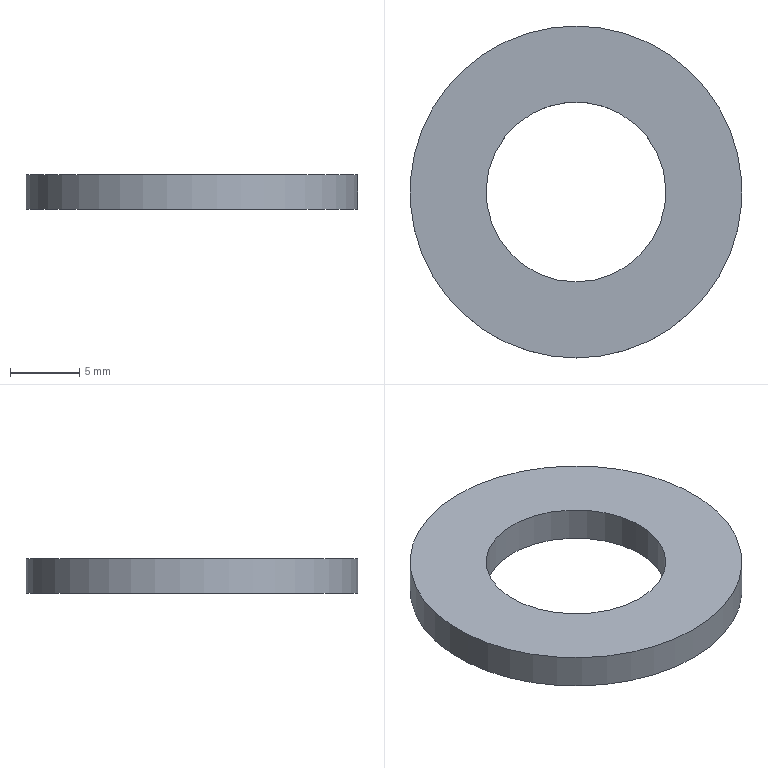Component | NX | 11 | 1 solid | 4 faces | box 24 x 24 x 2.5 mm | volume 799 mm3 | cylinder 2 | plane 2 | commonest cylinder face diameters 24 x1 13 x1
STEP:
#1=CARTESIAN_POINT('',(0.,0.,0.));
#2=DIRECTION('',(0.,0.,1.));
#3=DIRECTION('',(1.,0.,0.));
#4=AXIS2_PLACEMENT_3D('',#1,#2,#3);
#5=CARTESIAN_POINT('',(-30.,-42.,47.5));
#6=VERTEX_POINT('',#5);
#7=CARTESIAN_POINT('',(-30.,-30.,47.5));
#8=DIRECTION('',(0.,0.,1.));
#9=DIRECTION('',(0.00000005,-1.,0.));
#10=AXIS2_PLACEMENT_3D('',#7,#8,#9);
#11=CIRCLE('',#10,12.);
#12=CARTESIAN_POINT('',(-30.,-30.,47.5));
#13=DIRECTION('',(0.,0.,-1.));
#14=DIRECTION('',(-0.00000005,1.,0.));
#15=AXIS2_PLACEMENT_3D('',#12,#13,#14);
#16=CYLINDRICAL_SURFACE('',#15,12.);
#17=CARTESIAN_POINT('',(9.425,0.));
#18=DIRECTION('',(-1.,0.));
#19=VECTOR('',#18,1.);
#20=LINE('',#17,#19);
#21=(GEOMETRIC_REPRESENTATION_CONTEXT(2)PARAMETRIC_REPRESENTATION_CONTEXT()REPRESENTATION_CONTEXT('',''));
#22=DEFINITIONAL_REPRESENTATION('',(#20),#21);
#23=PCURVE('',#16,#22);
#24=CARTESIAN_POINT('',(-30.,-30.,47.5));
#25=DIRECTION('',(0.,0.,1.));
#26=DIRECTION('',(0.00000005,-1.,0.));
#27=AXIS2_PLACEMENT_3D('',#24,#25,#26);
#28=PLANE('',#27);
#29=CARTESIAN_POINT('',(0.,0.));
#30=DIRECTION('',(1.,-0.));
#31=AXIS2_PLACEMENT_2D('',#29,#30);
#32=CIRCLE('',#31,12.);
#33=(GEOMETRIC_REPRESENTATION_CONTEXT(2)PARAMETRIC_REPRESENTATION_CONTEXT()REPRESENTATION_CONTEXT('',''));
#34=DEFINITIONAL_REPRESENTATION('',(#32),#33);
#35=PCURVE('',#28,#34);
#36=SURFACE_CURVE('',#11,(#23,#35),.PCURVE_S1.);
#37=EDGE_CURVE('',#6,#6,#36,.T.);
#38=ORIENTED_EDGE('',*,*,#37,.F.);
#39=CARTESIAN_POINT('',(-30.,-42.,45.));
#40=VERTEX_POINT('',#39);
#41=CARTESIAN_POINT('',(-30.,-42.,47.5));
#42=CARTESIAN_POINT('',(-30.,-42.,45.));
#43=B_SPLINE_CURVE_WITH_KNOTS('',1,(#41,#42),.UNSPECIFIED.,.F.,.F.,(2,2),(0.,2.5),.PIECEWISE_BEZIER_KNOTS.);
#44=CARTESIAN_POINT('',(9.425,0.));
#45=DIRECTION('',(0.,1.));
#46=VECTOR('',#45,1.);
#47=LINE('',#44,#46);
#48=(GEOMETRIC_REPRESENTATION_CONTEXT(2)PARAMETRIC_REPRESENTATION_CONTEXT()REPRESENTATION_CONTEXT('',''));
#49=DEFINITIONAL_REPRESENTATION('',(#47),#48);
#50=PCURVE('',#16,#49);
#51=CARTESIAN_POINT('',(3.142,0.));
#52=DIRECTION('',(0.,1.));
#53=VECTOR('',#52,1.);
#54=LINE('',#51,#53);
#55=(GEOMETRIC_REPRESENTATION_CONTEXT(2)PARAMETRIC_REPRESENTATION_CONTEXT()REPRESENTATION_CONTEXT('',''));
#56=DEFINITIONAL_REPRESENTATION('',(#54),#55);
#57=PCURVE('',#16,#56);
#58=SEAM_CURVE('',#43,(#50,#57),.PCURVE_S1.);
#59=EDGE_CURVE('',#6,#40,#58,.T.);
#60=ORIENTED_EDGE('',*,*,#59,.T.);
#61=CARTESIAN_POINT('',(-30.,-30.,45.));
#62=DIRECTION('',(0.,0.,1.));
#63=DIRECTION('',(0.00000005,-1.,0.));
#64=AXIS2_PLACEMENT_3D('',#61,#62,#63);
#65=CIRCLE('',#64,12.);
#66=CARTESIAN_POINT('',(9.425,2.5));
#67=DIRECTION('',(-1.,0.));
#68=VECTOR('',#67,1.);
#69=LINE('',#66,#68);
#70=(GEOMETRIC_REPRESENTATION_CONTEXT(2)PARAMETRIC_REPRESENTATION_CONTEXT()REPRESENTATION_CONTEXT('',''));
#71=DEFINITIONAL_REPRESENTATION('',(#69),#70);
#72=PCURVE('',#16,#71);
#73=CARTESIAN_POINT('',(-30.,-30.,45.));
#74=DIRECTION('',(0.,0.,1.));
#75=DIRECTION('',(0.00000005,-1.,0.));
#76=AXIS2_PLACEMENT_3D('',#73,#74,#75);
#77=PLANE('',#76);
#78=CARTESIAN_POINT('',(0.,0.));
#79=DIRECTION('',(1.,-0.));
#80=AXIS2_PLACEMENT_2D('',#78,#79);
#81=CIRCLE('',#80,12.);
#82=(GEOMETRIC_REPRESENTATION_CONTEXT(2)PARAMETRIC_REPRESENTATION_CONTEXT()REPRESENTATION_CONTEXT('',''));
#83=DEFINITIONAL_REPRESENTATION('',(#81),#82);
#84=PCURVE('',#77,#83);
#85=SURFACE_CURVE('',#65,(#72,#84),.PCURVE_S1.);
#86=EDGE_CURVE('',#40,#40,#85,.T.);
#87=ORIENTED_EDGE('',*,*,#86,.T.);
#88=ORIENTED_EDGE('',*,*,#59,.F.);
#89=EDGE_LOOP('',(#38,#60,#87,#88));
#90=FACE_BOUND('',#89,.T.);
#91=ADVANCED_FACE('',(#90),#16,.T.);
#92=CARTESIAN_POINT('',(-30.,-36.5,47.5));
#93=VERTEX_POINT('',#92);
#94=CARTESIAN_POINT('',(-30.,-30.,47.5));
#95=DIRECTION('',(0.,0.,1.));
#96=DIRECTION('',(0.00000005,-1.,0.));
#97=AXIS2_PLACEMENT_3D('',#94,#95,#96);
#98=CIRCLE('',#97,6.5);
#99=CARTESIAN_POINT('',(-30.,-30.,47.5));
#100=DIRECTION('',(0.,0.,-1.));
#101=DIRECTION('',(-0.00000005,1.,0.));
#102=AXIS2_PLACEMENT_3D('',#99,#100,#101);
#103=CYLINDRICAL_SURFACE('',#102,6.5);
#104=CARTESIAN_POINT('',(9.425,0.));
#105=DIRECTION('',(-1.,0.));
#106=VECTOR('',#105,1.);
#107=LINE('',#104,#106);
#108=(GEOMETRIC_REPRESENTATION_CONTEXT(2)PARAMETRIC_REPRESENTATION_CONTEXT()REPRESENTATION_CONTEXT('',''));
#109=DEFINITIONAL_REPRESENTATION('',(#107),#108);
#110=PCURVE('',#103,#109);
#111=CARTESIAN_POINT('',(0.,0.));
#112=DIRECTION('',(1.,-0.));
#113=AXIS2_PLACEMENT_2D('',#111,#112);
#114=CIRCLE('',#113,6.5);
#115=(GEOMETRIC_REPRESENTATION_CONTEXT(2)PARAMETRIC_REPRESENTATION_CONTEXT()REPRESENTATION_CONTEXT('',''));
#116=DEFINITIONAL_REPRESENTATION('',(#114),#115);
#117=PCURVE('',#28,#116);
#118=SURFACE_CURVE('',#98,(#110,#117),.PCURVE_S1.);
#119=EDGE_CURVE('',#93,#93,#118,.T.);
#120=ORIENTED_EDGE('',*,*,#119,.F.);
#121=CARTESIAN_POINT('',(-30.,-36.5,45.));
#122=VERTEX_POINT('',#121);
#123=CARTESIAN_POINT('',(-30.,-36.5,47.5));
#124=CARTESIAN_POINT('',(-30.,-36.5,45.));
#125=B_SPLINE_CURVE_WITH_KNOTS('',1,(#123,#124),.UNSPECIFIED.,.F.,.F.,(2,2),(0.,2.5),.PIECEWISE_BEZIER_KNOTS.);
#126=CARTESIAN_POINT('',(9.425,0.));
#127=DIRECTION('',(0.,1.));
#128=VECTOR('',#127,1.);
#129=LINE('',#126,#128);
#130=(GEOMETRIC_REPRESENTATION_CONTEXT(2)PARAMETRIC_REPRESENTATION_CONTEXT()REPRESENTATION_CONTEXT('',''));
#131=DEFINITIONAL_REPRESENTATION('',(#129),#130);
#132=PCURVE('',#103,#131);
#133=CARTESIAN_POINT('',(3.142,0.));
#134=DIRECTION('',(0.,1.));
#135=VECTOR('',#134,1.);
#136=LINE('',#133,#135);
#137=(GEOMETRIC_REPRESENTATION_CONTEXT(2)PARAMETRIC_REPRESENTATION_CONTEXT()REPRESENTATION_CONTEXT('',''));
#138=DEFINITIONAL_REPRESENTATION('',(#136),#137);
#139=PCURVE('',#103,#138);
#140=SEAM_CURVE('',#125,(#132,#139),.PCURVE_S1.);
#141=EDGE_CURVE('',#93,#122,#140,.T.);
#142=ORIENTED_EDGE('',*,*,#141,.T.);
#143=CARTESIAN_POINT('',(-30.,-30.,45.));
#144=DIRECTION('',(0.,0.,1.));
#145=DIRECTION('',(0.00000005,-1.,0.));
#146=AXIS2_PLACEMENT_3D('',#143,#144,#145);
#147=CIRCLE('',#146,6.5);
#148=CARTESIAN_POINT('',(9.425,2.5));
#149=DIRECTION('',(-1.,0.));
#150=VECTOR('',#149,1.);
#151=LINE('',#148,#150);
#152=(GEOMETRIC_REPRESENTATION_CONTEXT(2)PARAMETRIC_REPRESENTATION_CONTEXT()REPRESENTATION_CONTEXT('',''));
#153=DEFINITIONAL_REPRESENTATION('',(#151),#152);
#154=PCURVE('',#103,#153);
#155=CARTESIAN_POINT('',(0.,0.));
#156=DIRECTION('',(1.,-0.));
#157=AXIS2_PLACEMENT_2D('',#155,#156);
#158=CIRCLE('',#157,6.5);
#159=(GEOMETRIC_REPRESENTATION_CONTEXT(2)PARAMETRIC_REPRESENTATION_CONTEXT()REPRESENTATION_CONTEXT('',''));
#160=DEFINITIONAL_REPRESENTATION('',(#158),#159);
#161=PCURVE('',#77,#160);
#162=SURFACE_CURVE('',#147,(#154,#161),.PCURVE_S1.);
#163=EDGE_CURVE('',#122,#122,#162,.T.);
#164=ORIENTED_EDGE('',*,*,#163,.T.);
#165=ORIENTED_EDGE('',*,*,#141,.F.);
#166=EDGE_LOOP('',(#120,#142,#164,#165));
#167=FACE_BOUND('',#166,.F.);
#168=ADVANCED_FACE('',(#167),#103,.F.);
#169=ORIENTED_EDGE('',*,*,#37,.T.);
#170=EDGE_LOOP('',(#169));
#171=FACE_BOUND('',#170,.T.);
#172=ORIENTED_EDGE('',*,*,#119,.F.);
#173=EDGE_LOOP('',(#172));
#174=FACE_BOUND('',#173,.T.);
#175=ADVANCED_FACE('',(#171,#174),#28,.T.);
#176=ORIENTED_EDGE('',*,*,#86,.F.);
#177=EDGE_LOOP('',(#176));
#178=FACE_BOUND('',#177,.T.);
#179=ORIENTED_EDGE('',*,*,#163,.T.);
#180=EDGE_LOOP('',(#179));
#181=FACE_BOUND('',#180,.T.);
#182=ADVANCED_FACE('',(#178,#181),#77,.F.);
#183=CLOSED_SHELL('',(#91,#168,#175,#182));
#184=MANIFOLD_SOLID_BREP('',#183);
#185=(LENGTH_UNIT()NAMED_UNIT(*)SI_UNIT(.MILLI.,.METRE.));
#186=UNCERTAINTY_MEASURE_WITH_UNIT(LENGTH_MEASURE(0.00001),#185,'','');
#187=(NAMED_UNIT(*)PLANE_ANGLE_UNIT()SI_UNIT($,.RADIAN.));
#188=(NAMED_UNIT(*)SI_UNIT($,.STERADIAN.)SOLID_ANGLE_UNIT());
#189=(GEOMETRIC_REPRESENTATION_CONTEXT(3)GLOBAL_UNCERTAINTY_ASSIGNED_CONTEXT((#186))GLOBAL_UNIT_ASSIGNED_CONTEXT((#185,#187,#188))REPRESENTATION_CONTEXT('',''));
#190=ADVANCED_BREP_SHAPE_REPRESENTATION('',(#4,#184),#189);